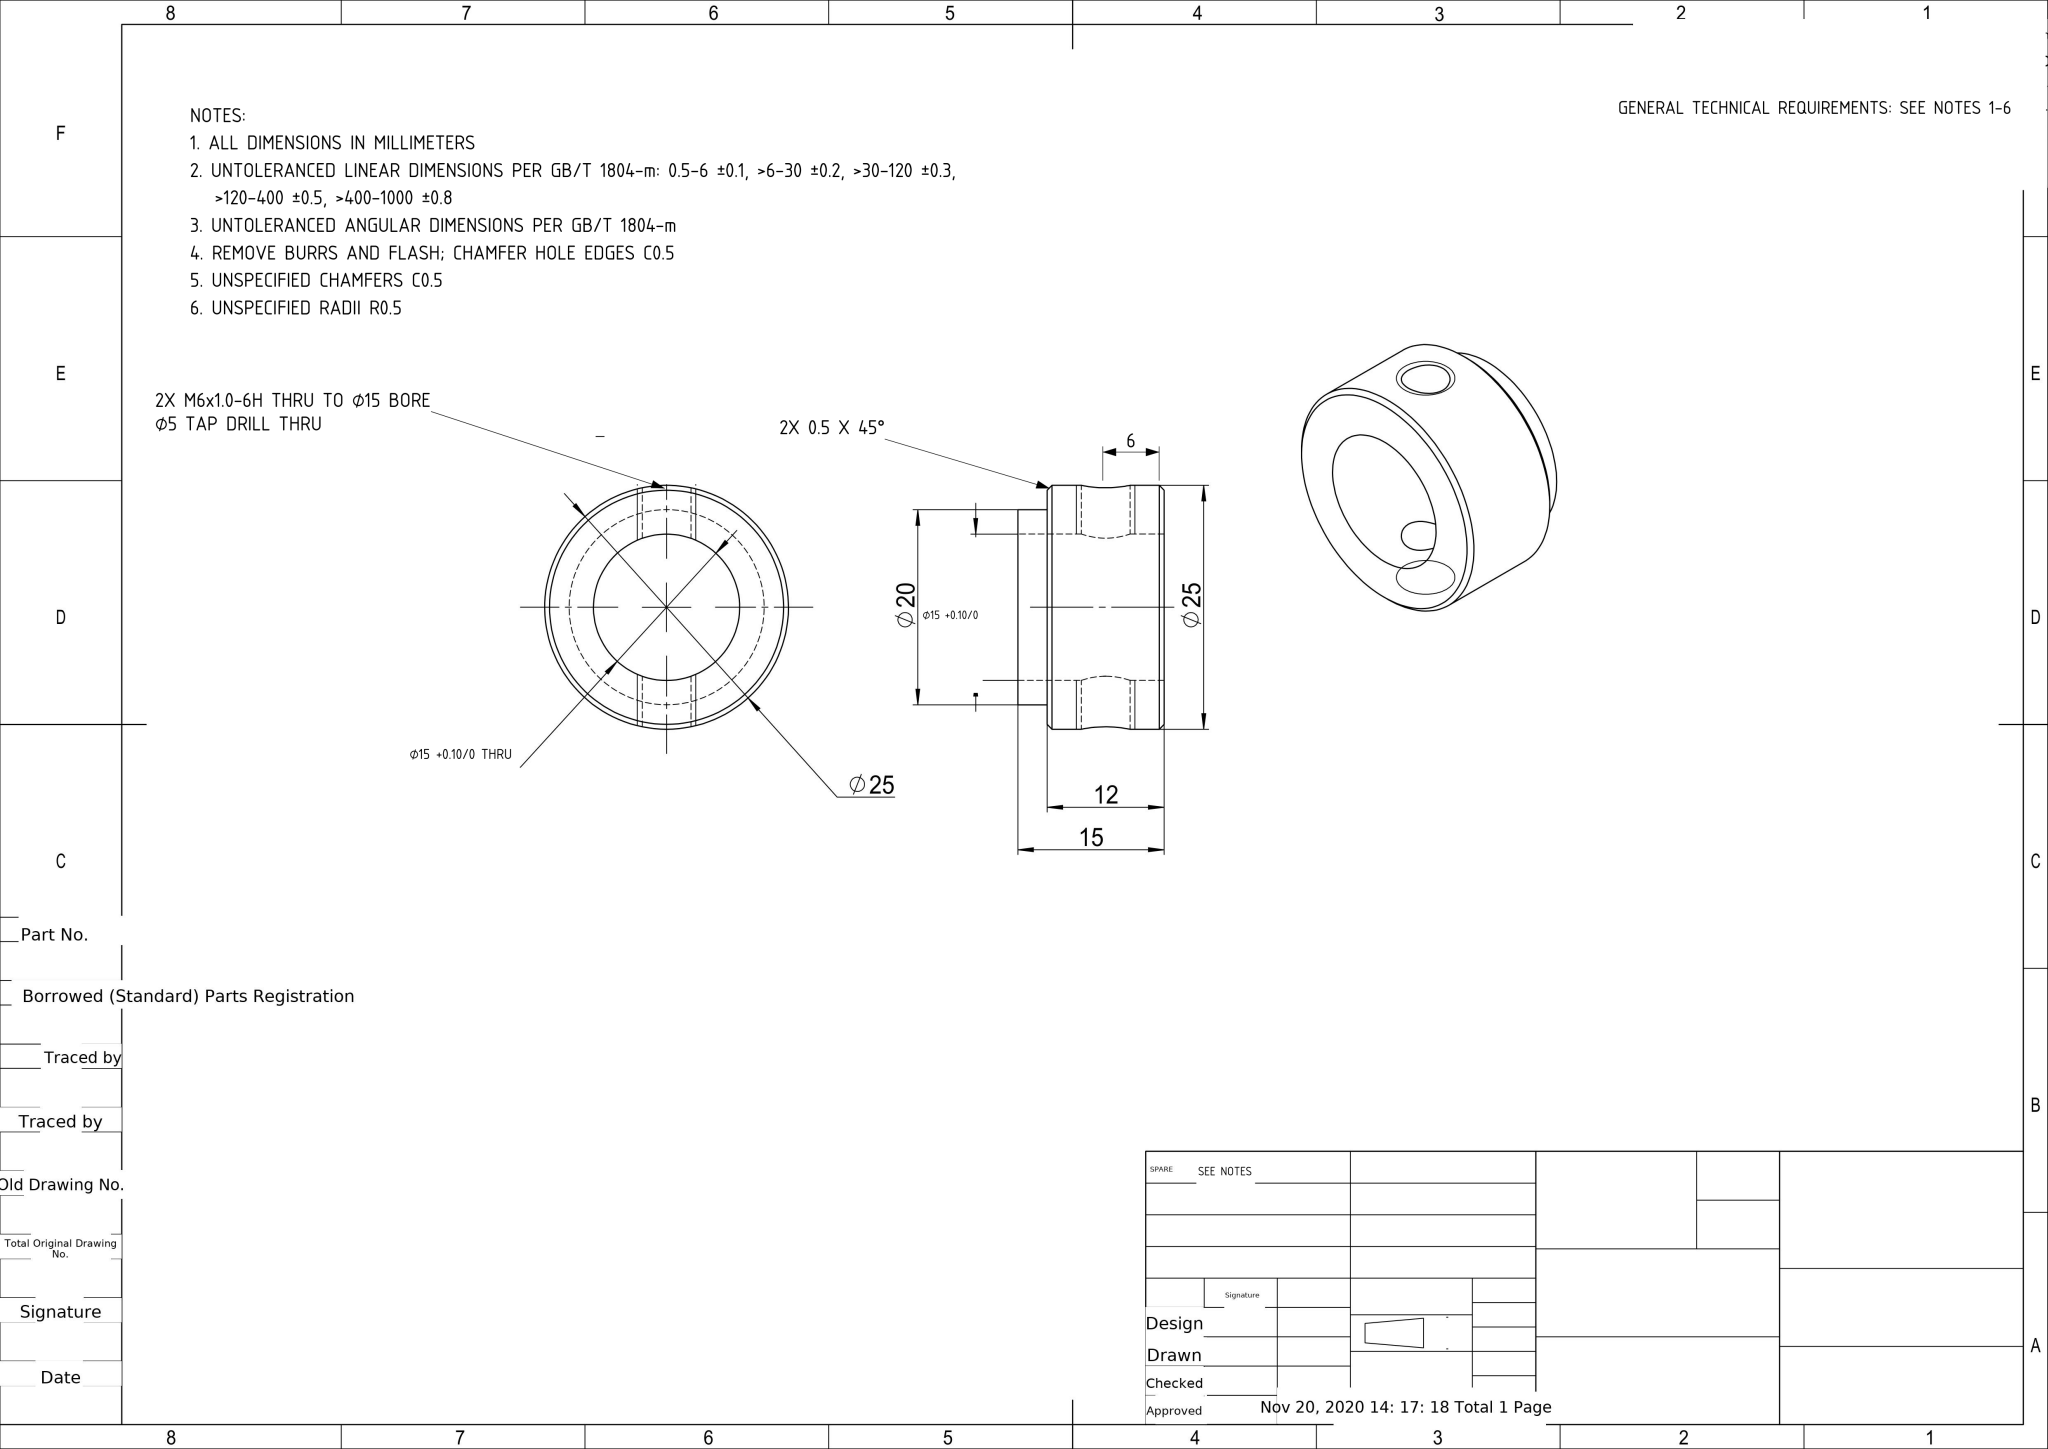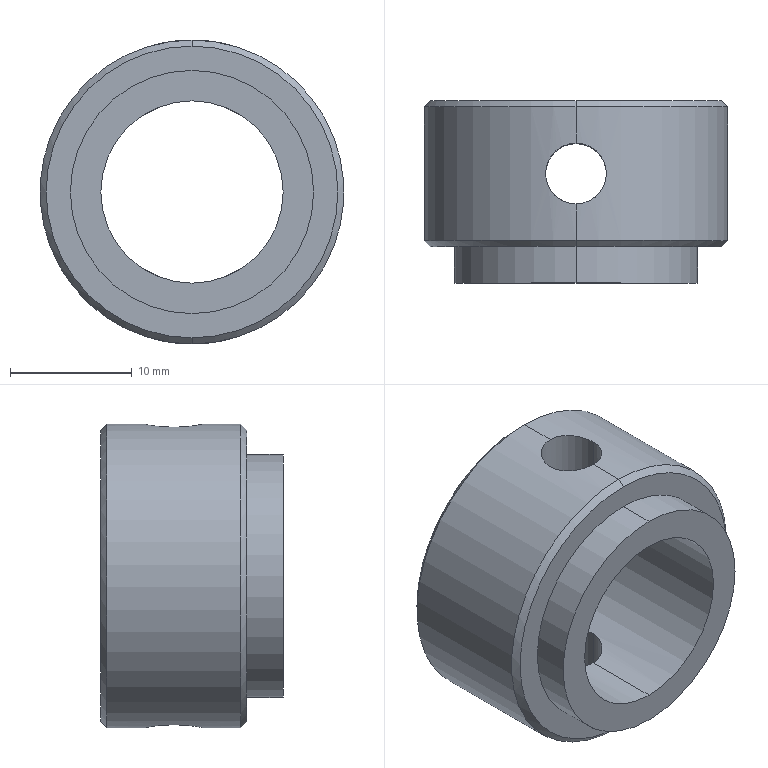Part | NX | mm | 1 solid | 17 faces | box 25 x 15 x 25 mm | volume 3965 mm3 | cylinder 10 | cone 4 | plane 3 | commonest cylinder face diameters 5 x4 20 x2 15 x2 25 x2